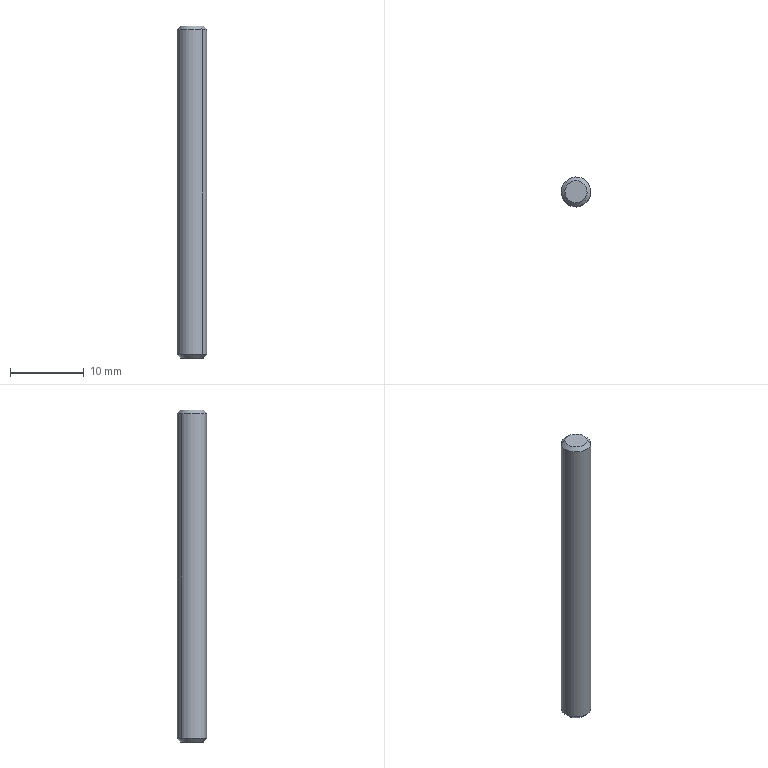Component | SolidWorks | TapeGuideRollerAxis-1 | 1 solid | 8 faces | box 4 x 4 x 45 mm | volume 563 mm3 | cone 4 | cylinder 2 | plane 2 | commonest cylinder face diameters 4 x2
STEP:
#1=COLOUR_RGB('',0.7922,0.8196,0.9333);
#2=FILL_AREA_STYLE_COLOUR('',#1);
#3=FILL_AREA_STYLE('',(#2));
#4=SURFACE_STYLE_FILL_AREA(#3);
#5=SURFACE_SIDE_STYLE('',(#4));
#6=SURFACE_STYLE_USAGE(.BOTH.,#5);
#7=PRESENTATION_STYLE_ASSIGNMENT((#6));
#8=CARTESIAN_POINT('',(-6.374,5.051,2.187));
#9=VERTEX_POINT('',#8);
#10=CARTESIAN_POINT('',(-6.264,4.939,2.187));
#11=VERTEX_POINT('',#10);
#12=CARTESIAN_POINT('',(-6.319,4.995,2.187));
#13=DIRECTION('',(-0.,0.,-1.));
#14=DIRECTION('',(-0.7017,0.7124,0.));
#15=AXIS2_PLACEMENT_3D('',#12,#13,#14);
#16=CIRCLE('',#15,0.07874);
#17=EDGE_CURVE('',#9,#11,#16,.T.);
#18=ORIENTED_EDGE('',*,*,#17,.T.);
#19=CARTESIAN_POINT('',(-6.264,4.939,0.4544));
#20=VERTEX_POINT('',#19);
#21=CARTESIAN_POINT('',(-6.264,4.939,2.206));
#22=DIRECTION('',(-0.,0.,-1.));
#23=VECTOR('',#22,39.37);
#24=LINE('',#21,#23);
#25=EDGE_CURVE('',#11,#20,#24,.T.);
#26=ORIENTED_EDGE('',*,*,#25,.T.);
#27=CARTESIAN_POINT('',(-6.374,5.051,0.4544));
#28=VERTEX_POINT('',#27);
#29=CARTESIAN_POINT('',(-6.319,4.995,0.4544));
#30=DIRECTION('',(0.,-0.,1.));
#31=DIRECTION('',(-0.7017,0.7124,0.));
#32=AXIS2_PLACEMENT_3D('',#29,#30,#31);
#33=CIRCLE('',#32,0.07874);
#34=EDGE_CURVE('',#20,#28,#33,.T.);
#35=ORIENTED_EDGE('',*,*,#34,.T.);
#36=CARTESIAN_POINT('',(-6.374,5.051,2.206));
#37=DIRECTION('',(-0.,0.,-1.));
#38=VECTOR('',#37,39.37);
#39=LINE('',#36,#38);
#40=EDGE_CURVE('',#9,#28,#39,.T.);
#41=ORIENTED_EDGE('',*,*,#40,.F.);
#42=EDGE_LOOP('',(#18,#26,#35,#41));
#43=FACE_OUTER_BOUND('',#42,.T.);
#44=CARTESIAN_POINT('',(-6.319,4.995,2.206));
#45=DIRECTION('',(-0.,0.,-1.));
#46=DIRECTION('',(-0.7017,0.7124,0.));
#47=AXIS2_PLACEMENT_3D('',#44,#45,#46);
#48=CYLINDRICAL_SURFACE('',#47,0.07874);
#49=ADVANCED_FACE('',(#43),#48,.T.);
#50=CARTESIAN_POINT('',(-6.277,4.953,0.4347));
#51=VERTEX_POINT('',#50);
#52=CARTESIAN_POINT('',(-6.36,5.037,0.4347));
#53=VERTEX_POINT('',#52);
#54=CARTESIAN_POINT('',(-6.319,4.995,0.4347));
#55=DIRECTION('',(0.,-0.,1.));
#56=DIRECTION('',(0.7017,-0.7124,0.));
#57=AXIS2_PLACEMENT_3D('',#54,#55,#56);
#58=CIRCLE('',#57,0.05906);
#59=EDGE_CURVE('',#51,#53,#58,.T.);
#60=ORIENTED_EDGE('',*,*,#59,.T.);
#61=CARTESIAN_POINT('',(-6.374,5.051,0.4544));
#62=DIRECTION('',(-0.4962,0.5038,0.7071));
#63=VECTOR('',#62,39.37);
#64=LINE('',#61,#63);
#65=EDGE_CURVE('',#53,#28,#64,.T.);
#66=ORIENTED_EDGE('',*,*,#65,.T.);
#67=ORIENTED_EDGE('',*,*,#34,.F.);
#68=CARTESIAN_POINT('',(-6.264,4.939,0.4544));
#69=DIRECTION('',(0.4962,-0.5038,0.7071));
#70=VECTOR('',#69,39.37);
#71=LINE('',#68,#70);
#72=EDGE_CURVE('',#51,#20,#71,.T.);
#73=ORIENTED_EDGE('',*,*,#72,.F.);
#74=EDGE_LOOP('',(#60,#66,#67,#73));
#75=FACE_OUTER_BOUND('',#74,.T.);
#76=CARTESIAN_POINT('',(-6.319,4.995,0.4544));
#77=DIRECTION('',(0.,-0.,1.));
#78=DIRECTION('',(0.7017,-0.7124,0.));
#79=AXIS2_PLACEMENT_3D('',#76,#77,#78);
#80=CONICAL_SURFACE('',#79,0.07874,0.7854);
#81=ADVANCED_FACE('',(#75),#80,.T.);
#82=CARTESIAN_POINT('',(-6.36,5.037,2.206));
#83=VERTEX_POINT('',#82);
#84=CARTESIAN_POINT('',(-6.277,4.953,2.206));
#85=VERTEX_POINT('',#84);
#86=CARTESIAN_POINT('',(-6.319,4.995,2.206));
#87=DIRECTION('',(-0.,0.,-1.));
#88=DIRECTION('',(-0.7017,0.7124,0.));
#89=AXIS2_PLACEMENT_3D('',#86,#87,#88);
#90=CIRCLE('',#89,0.05906);
#91=EDGE_CURVE('',#83,#85,#90,.T.);
#92=ORIENTED_EDGE('',*,*,#91,.T.);
#93=CARTESIAN_POINT('',(-6.264,4.939,2.187));
#94=DIRECTION('',(0.4962,-0.5038,-0.7071));
#95=VECTOR('',#94,39.37);
#96=LINE('',#93,#95);
#97=EDGE_CURVE('',#85,#11,#96,.T.);
#98=ORIENTED_EDGE('',*,*,#97,.T.);
#99=ORIENTED_EDGE('',*,*,#17,.F.);
#100=CARTESIAN_POINT('',(-6.374,5.051,2.187));
#101=DIRECTION('',(-0.4962,0.5038,-0.7071));
#102=VECTOR('',#101,39.37);
#103=LINE('',#100,#102);
#104=EDGE_CURVE('',#83,#9,#103,.T.);
#105=ORIENTED_EDGE('',*,*,#104,.F.);
#106=EDGE_LOOP('',(#92,#98,#99,#105));
#107=FACE_OUTER_BOUND('',#106,.T.);
#108=CARTESIAN_POINT('',(-6.319,4.995,2.187));
#109=DIRECTION('',(-0.,0.,-1.));
#110=DIRECTION('',(-0.7017,0.7124,0.));
#111=AXIS2_PLACEMENT_3D('',#108,#109,#110);
#112=CONICAL_SURFACE('',#111,0.07874,0.7854);
#113=ADVANCED_FACE('',(#107),#112,.T.);
#114=ORIENTED_EDGE('',*,*,#25,.F.);
#115=CARTESIAN_POINT('',(-6.319,4.995,2.187));
#116=DIRECTION('',(-0.,0.,-1.));
#117=DIRECTION('',(-0.7017,0.7124,0.));
#118=AXIS2_PLACEMENT_3D('',#115,#116,#117);
#119=CIRCLE('',#118,0.07874);
#120=EDGE_CURVE('',#11,#9,#119,.T.);
#121=ORIENTED_EDGE('',*,*,#120,.T.);
#122=ORIENTED_EDGE('',*,*,#40,.T.);
#123=CARTESIAN_POINT('',(-6.319,4.995,0.4544));
#124=DIRECTION('',(0.,-0.,1.));
#125=DIRECTION('',(-0.7017,0.7124,0.));
#126=AXIS2_PLACEMENT_3D('',#123,#124,#125);
#127=CIRCLE('',#126,0.07874);
#128=EDGE_CURVE('',#28,#20,#127,.T.);
#129=ORIENTED_EDGE('',*,*,#128,.T.);
#130=EDGE_LOOP('',(#114,#121,#122,#129));
#131=FACE_OUTER_BOUND('',#130,.T.);
#132=CARTESIAN_POINT('',(-6.319,4.995,2.206));
#133=DIRECTION('',(-0.,0.,-1.));
#134=DIRECTION('',(-0.7017,0.7124,0.));
#135=AXIS2_PLACEMENT_3D('',#132,#133,#134);
#136=CYLINDRICAL_SURFACE('',#135,0.07874);
#137=ADVANCED_FACE('',(#131),#136,.T.);
#138=ORIENTED_EDGE('',*,*,#65,.F.);
#139=CARTESIAN_POINT('',(-6.319,4.995,0.4347));
#140=DIRECTION('',(0.,-0.,1.));
#141=DIRECTION('',(0.7017,-0.7124,0.));
#142=AXIS2_PLACEMENT_3D('',#139,#140,#141);
#143=CIRCLE('',#142,0.05906);
#144=EDGE_CURVE('',#53,#51,#143,.T.);
#145=ORIENTED_EDGE('',*,*,#144,.T.);
#146=ORIENTED_EDGE('',*,*,#72,.T.);
#147=ORIENTED_EDGE('',*,*,#128,.F.);
#148=EDGE_LOOP('',(#138,#145,#146,#147));
#149=FACE_OUTER_BOUND('',#148,.T.);
#150=CARTESIAN_POINT('',(-6.319,4.995,0.4544));
#151=DIRECTION('',(0.,-0.,1.));
#152=DIRECTION('',(0.7017,-0.7124,0.));
#153=AXIS2_PLACEMENT_3D('',#150,#151,#152);
#154=CONICAL_SURFACE('',#153,0.07874,0.7854);
#155=ADVANCED_FACE('',(#149),#154,.T.);
#156=ORIENTED_EDGE('',*,*,#97,.F.);
#157=CARTESIAN_POINT('',(-6.319,4.995,2.206));
#158=DIRECTION('',(-0.,0.,-1.));
#159=DIRECTION('',(-0.7017,0.7124,0.));
#160=AXIS2_PLACEMENT_3D('',#157,#158,#159);
#161=CIRCLE('',#160,0.05906);
#162=EDGE_CURVE('',#85,#83,#161,.T.);
#163=ORIENTED_EDGE('',*,*,#162,.T.);
#164=ORIENTED_EDGE('',*,*,#104,.T.);
#165=ORIENTED_EDGE('',*,*,#120,.F.);
#166=EDGE_LOOP('',(#156,#163,#164,#165));
#167=FACE_OUTER_BOUND('',#166,.T.);
#168=CARTESIAN_POINT('',(-6.319,4.995,2.187));
#169=DIRECTION('',(-0.,0.,-1.));
#170=DIRECTION('',(-0.7017,0.7124,0.));
#171=AXIS2_PLACEMENT_3D('',#168,#169,#170);
#172=CONICAL_SURFACE('',#171,0.07874,0.7854);
#173=ADVANCED_FACE('',(#167),#172,.T.);
#174=ORIENTED_EDGE('',*,*,#59,.F.);
#175=ORIENTED_EDGE('',*,*,#144,.F.);
#176=EDGE_LOOP('',(#174,#175));
#177=FACE_OUTER_BOUND('',#176,.T.);
#178=CARTESIAN_POINT('',(-6.319,4.995,0.4347));
#179=DIRECTION('',(0.,-0.,1.));
#180=DIRECTION('',(0.7017,-0.7124,-0.));
#181=AXIS2_PLACEMENT_3D('',#178,#179,#180);
#182=PLANE('',#181);
#183=ADVANCED_FACE('',(#177),#182,.F.);
#184=ORIENTED_EDGE('',*,*,#91,.F.);
#185=ORIENTED_EDGE('',*,*,#162,.F.);
#186=EDGE_LOOP('',(#184,#185));
#187=FACE_OUTER_BOUND('',#186,.T.);
#188=CARTESIAN_POINT('',(-6.319,4.995,2.206));
#189=DIRECTION('',(0.,-0.,1.));
#190=DIRECTION('',(0.7017,-0.7124,-0.));
#191=AXIS2_PLACEMENT_3D('',#188,#189,#190);
#192=PLANE('',#191);
#193=ADVANCED_FACE('',(#187),#192,.T.);
#194=CLOSED_SHELL('',(#49,#81,#113,#137,#155,#173,#183,#193));
#195=MANIFOLD_SOLID_BREP('',#194);
#196=STYLED_ITEM('',(#7),#195);
#197=(LENGTH_UNIT()NAMED_UNIT(*)SI_UNIT($,.METRE.));
#198=LENGTH_MEASURE_WITH_UNIT(LENGTH_MEASURE(0.0254),#197);
#199=DIMENSIONAL_EXPONENTS(1.,0.,0.,0.,0.,0.,0.);
#200=(CONVERSION_BASED_UNIT('',#198)LENGTH_UNIT()NAMED_UNIT(#199));
#201=UNCERTAINTY_MEASURE_WITH_UNIT(LENGTH_MEASURE(0.00001),#200,'','');
#202=(NAMED_UNIT(*)PLANE_ANGLE_UNIT()SI_UNIT($,.RADIAN.));
#203=(NAMED_UNIT(*)SI_UNIT($,.STERADIAN.)SOLID_ANGLE_UNIT());
#204=(GEOMETRIC_REPRESENTATION_CONTEXT(3)GLOBAL_UNCERTAINTY_ASSIGNED_CONTEXT((#201))GLOBAL_UNIT_ASSIGNED_CONTEXT((#200,#202,#203))REPRESENTATION_CONTEXT('',''));
#205=MECHANICAL_DESIGN_GEOMETRIC_PRESENTATION_REPRESENTATION('',(#196),#204);
#206=PRESENTATION_LAYER_ASSIGNMENT('','',(#196));
#207=CARTESIAN_POINT('',(0.,0.,0.));
#208=DIRECTION('',(0.,0.,1.));
#209=DIRECTION('',(1.,0.,0.));
#210=AXIS2_PLACEMENT_3D('',#207,#208,#209);
#211=(LENGTH_UNIT()NAMED_UNIT(*)SI_UNIT($,.METRE.));
#212=LENGTH_MEASURE_WITH_UNIT(LENGTH_MEASURE(0.0254),#211);
#213=DIMENSIONAL_EXPONENTS(1.,0.,0.,0.,0.,0.,0.);
#214=(CONVERSION_BASED_UNIT('',#212)LENGTH_UNIT()NAMED_UNIT(#213));
#215=UNCERTAINTY_MEASURE_WITH_UNIT(LENGTH_MEASURE(0.00001),#214,'','');
#216=(NAMED_UNIT(*)PLANE_ANGLE_UNIT()SI_UNIT($,.RADIAN.));
#217=(NAMED_UNIT(*)SI_UNIT($,.STERADIAN.)SOLID_ANGLE_UNIT());
#218=(GEOMETRIC_REPRESENTATION_CONTEXT(3)GLOBAL_UNCERTAINTY_ASSIGNED_CONTEXT((#215))GLOBAL_UNIT_ASSIGNED_CONTEXT((#214,#216,#217))REPRESENTATION_CONTEXT('',''));
#219=ADVANCED_BREP_SHAPE_REPRESENTATION('',(#195,#210),#218);